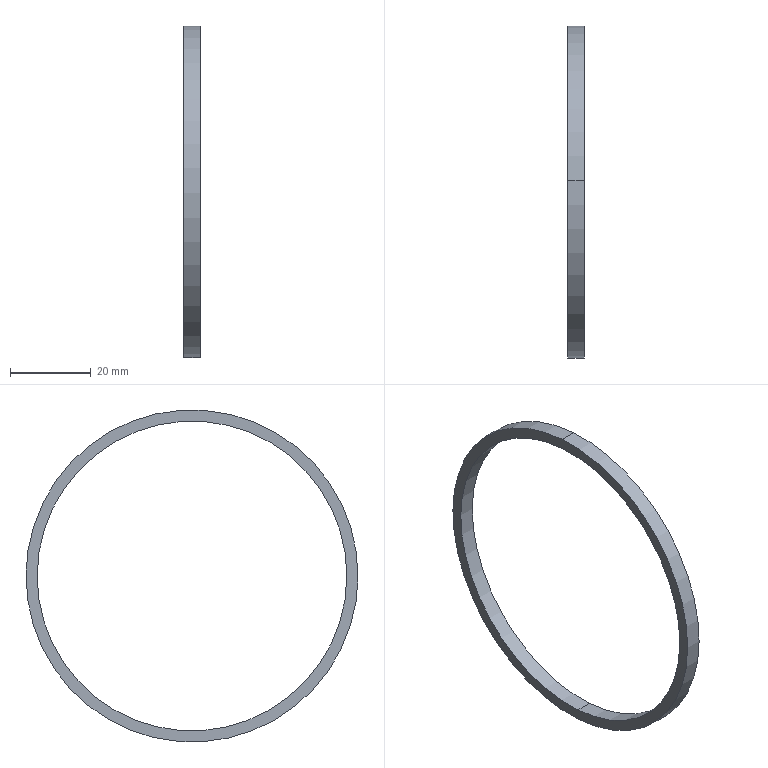Component | SolidWorks | 2018SOLIDWORKS1000000506-1 | 1 solid | 6 faces | box 4 x 82 x 82 mm | volume 2739 mm3 | cylinder 4 | plane 2 | commonest cylinder face diameters 76.5 x2 82 x2 | material 201
build123d program:
from build123d import *

# Parameters (mm, degrees)
SKETCH1_R           = 41
SKETCH1_R_2         = 38.25
BOSS_EXTRUDE1_DEPTH = 4


with BuildPart() as part:
    # Sketch1 → Boss-Extrude1 (new body)
    with BuildSketch(Plane.XY):
        Circle(SKETCH1_R)
        Circle(SKETCH1_R_2, mode=Mode.SUBTRACT)
    extrude(amount=BOSS_EXTRUDE1_DEPTH)


solid = part.part

# Placed as in the assembly
solid = solid.moved(Location((2.716, -95.825, 207.018), (0, 90, 0)))
STEP:
#1=COLOUR_RGB('',0.7922,0.8196,0.9333);
#2=FILL_AREA_STYLE_COLOUR('',#1);
#3=FILL_AREA_STYLE('',(#2));
#4=SURFACE_STYLE_FILL_AREA(#3);
#5=SURFACE_SIDE_STYLE('',(#4));
#6=SURFACE_STYLE_USAGE(.BOTH.,#5);
#7=PRESENTATION_STYLE_ASSIGNMENT((#6));
#8=CARTESIAN_POINT('',(0.2644,-3.668,9.653));
#9=VERTEX_POINT('',#8);
#10=CARTESIAN_POINT('',(0.2644,-3.878,6.648));
#11=VERTEX_POINT('',#10);
#12=CARTESIAN_POINT('',(0.2644,-3.773,8.15));
#13=DIRECTION('',(1.,0.,-0.));
#14=DIRECTION('',(-0.,-0.06975,-0.9976));
#15=AXIS2_PLACEMENT_3D('',#12,#13,#14);
#16=CIRCLE('',#15,1.506);
#17=EDGE_CURVE('',#9,#11,#16,.T.);
#18=ORIENTED_EDGE('',*,*,#17,.T.);
#19=CARTESIAN_POINT('',(0.1069,-3.878,6.648));
#20=VERTEX_POINT('',#19);
#21=CARTESIAN_POINT('',(0.2644,-3.878,6.648));
#22=DIRECTION('',(-1.,-0.,0.));
#23=VECTOR('',#22,39.37);
#24=LINE('',#21,#23);
#25=EDGE_CURVE('',#11,#20,#24,.T.);
#26=ORIENTED_EDGE('',*,*,#25,.T.);
#27=CARTESIAN_POINT('',(0.1069,-3.668,9.653));
#28=VERTEX_POINT('',#27);
#29=CARTESIAN_POINT('',(0.1069,-3.773,8.15));
#30=DIRECTION('',(1.,0.,-0.));
#31=DIRECTION('',(-0.,-0.06975,-0.9976));
#32=AXIS2_PLACEMENT_3D('',#29,#30,#31);
#33=CIRCLE('',#32,1.506);
#34=EDGE_CURVE('',#28,#20,#33,.T.);
#35=ORIENTED_EDGE('',*,*,#34,.F.);
#36=CARTESIAN_POINT('',(0.2644,-3.668,9.653));
#37=DIRECTION('',(-1.,-0.,0.));
#38=VECTOR('',#37,39.37);
#39=LINE('',#36,#38);
#40=EDGE_CURVE('',#9,#28,#39,.T.);
#41=ORIENTED_EDGE('',*,*,#40,.F.);
#42=EDGE_LOOP('',(#18,#26,#35,#41));
#43=FACE_OUTER_BOUND('',#42,.T.);
#44=CARTESIAN_POINT('',(0.2644,-3.773,8.15));
#45=DIRECTION('',(-1.,-0.,0.));
#46=DIRECTION('',(0.,0.06975,0.9976));
#47=AXIS2_PLACEMENT_3D('',#44,#45,#46);
#48=CYLINDRICAL_SURFACE('',#47,1.506);
#49=ADVANCED_FACE('',(#43),#48,.F.);
#50=CARTESIAN_POINT('',(0.2644,-3.885,6.54));
#51=VERTEX_POINT('',#50);
#52=CARTESIAN_POINT('',(0.2644,-3.66,9.761));
#53=VERTEX_POINT('',#52);
#54=CARTESIAN_POINT('',(0.2644,-3.773,8.15));
#55=DIRECTION('',(1.,0.,-0.));
#56=DIRECTION('',(-0.,-0.06975,-0.9976));
#57=AXIS2_PLACEMENT_3D('',#54,#55,#56);
#58=CIRCLE('',#57,1.614);
#59=EDGE_CURVE('',#51,#53,#58,.T.);
#60=ORIENTED_EDGE('',*,*,#59,.F.);
#61=CARTESIAN_POINT('',(0.1069,-3.885,6.54));
#62=VERTEX_POINT('',#61);
#63=CARTESIAN_POINT('',(0.2644,-3.885,6.54));
#64=DIRECTION('',(-1.,-0.,0.));
#65=VECTOR('',#64,39.37);
#66=LINE('',#63,#65);
#67=EDGE_CURVE('',#51,#62,#66,.T.);
#68=ORIENTED_EDGE('',*,*,#67,.T.);
#69=CARTESIAN_POINT('',(0.1069,-3.66,9.761));
#70=VERTEX_POINT('',#69);
#71=CARTESIAN_POINT('',(0.1069,-3.773,8.15));
#72=DIRECTION('',(1.,0.,-0.));
#73=DIRECTION('',(-0.,-0.06975,-0.9976));
#74=AXIS2_PLACEMENT_3D('',#71,#72,#73);
#75=CIRCLE('',#74,1.614);
#76=EDGE_CURVE('',#62,#70,#75,.T.);
#77=ORIENTED_EDGE('',*,*,#76,.T.);
#78=CARTESIAN_POINT('',(0.2644,-3.66,9.761));
#79=DIRECTION('',(-1.,-0.,0.));
#80=VECTOR('',#79,39.37);
#81=LINE('',#78,#80);
#82=EDGE_CURVE('',#53,#70,#81,.T.);
#83=ORIENTED_EDGE('',*,*,#82,.F.);
#84=EDGE_LOOP('',(#60,#68,#77,#83));
#85=FACE_OUTER_BOUND('',#84,.T.);
#86=CARTESIAN_POINT('',(0.2644,-3.773,8.15));
#87=DIRECTION('',(-1.,-0.,0.));
#88=DIRECTION('',(0.,0.06975,0.9976));
#89=AXIS2_PLACEMENT_3D('',#86,#87,#88);
#90=CYLINDRICAL_SURFACE('',#89,1.614);
#91=ADVANCED_FACE('',(#85),#90,.T.);
#92=CARTESIAN_POINT('',(0.2644,-3.773,8.15));
#93=DIRECTION('',(1.,0.,-0.));
#94=DIRECTION('',(-0.,-0.06975,-0.9976));
#95=AXIS2_PLACEMENT_3D('',#92,#93,#94);
#96=CIRCLE('',#95,1.614);
#97=EDGE_CURVE('',#53,#51,#96,.T.);
#98=ORIENTED_EDGE('',*,*,#97,.T.);
#99=ORIENTED_EDGE('',*,*,#59,.T.);
#100=EDGE_LOOP('',(#98,#99));
#101=FACE_OUTER_BOUND('',#100,.T.);
#102=ORIENTED_EDGE('',*,*,#17,.F.);
#103=CARTESIAN_POINT('',(0.2644,-3.773,8.15));
#104=DIRECTION('',(1.,0.,-0.));
#105=DIRECTION('',(-0.,-0.06975,-0.9976));
#106=AXIS2_PLACEMENT_3D('',#103,#104,#105);
#107=CIRCLE('',#106,1.506);
#108=EDGE_CURVE('',#11,#9,#107,.T.);
#109=ORIENTED_EDGE('',*,*,#108,.F.);
#110=EDGE_LOOP('',(#102,#109));
#111=FACE_BOUND('',#110,.T.);
#112=CARTESIAN_POINT('',(0.2644,-3.773,8.15));
#113=DIRECTION('',(1.,0.,-0.));
#114=DIRECTION('',(-0.,-0.06975,-0.9976));
#115=AXIS2_PLACEMENT_3D('',#112,#113,#114);
#116=PLANE('',#115);
#117=ADVANCED_FACE('',(#101,#111),#116,.T.);
#118=CARTESIAN_POINT('',(0.1069,-3.773,8.15));
#119=DIRECTION('',(1.,0.,-0.));
#120=DIRECTION('',(-0.,-0.06975,-0.9976));
#121=AXIS2_PLACEMENT_3D('',#118,#119,#120);
#122=CIRCLE('',#121,1.614);
#123=EDGE_CURVE('',#70,#62,#122,.T.);
#124=ORIENTED_EDGE('',*,*,#123,.F.);
#125=ORIENTED_EDGE('',*,*,#76,.F.);
#126=EDGE_LOOP('',(#124,#125));
#127=FACE_OUTER_BOUND('',#126,.T.);
#128=ORIENTED_EDGE('',*,*,#34,.T.);
#129=CARTESIAN_POINT('',(0.1069,-3.773,8.15));
#130=DIRECTION('',(1.,0.,-0.));
#131=DIRECTION('',(-0.,-0.06975,-0.9976));
#132=AXIS2_PLACEMENT_3D('',#129,#130,#131);
#133=CIRCLE('',#132,1.506);
#134=EDGE_CURVE('',#20,#28,#133,.T.);
#135=ORIENTED_EDGE('',*,*,#134,.T.);
#136=EDGE_LOOP('',(#128,#135));
#137=FACE_BOUND('',#136,.T.);
#138=CARTESIAN_POINT('',(0.1069,-3.773,8.15));
#139=DIRECTION('',(1.,0.,-0.));
#140=DIRECTION('',(-0.,-0.06975,-0.9976));
#141=AXIS2_PLACEMENT_3D('',#138,#139,#140);
#142=PLANE('',#141);
#143=ADVANCED_FACE('',(#127,#137),#142,.F.);
#144=ORIENTED_EDGE('',*,*,#67,.F.);
#145=ORIENTED_EDGE('',*,*,#97,.F.);
#146=ORIENTED_EDGE('',*,*,#82,.T.);
#147=ORIENTED_EDGE('',*,*,#123,.T.);
#148=EDGE_LOOP('',(#144,#145,#146,#147));
#149=FACE_OUTER_BOUND('',#148,.T.);
#150=CARTESIAN_POINT('',(0.2644,-3.773,8.15));
#151=DIRECTION('',(-1.,-0.,0.));
#152=DIRECTION('',(0.,0.06975,0.9976));
#153=AXIS2_PLACEMENT_3D('',#150,#151,#152);
#154=CYLINDRICAL_SURFACE('',#153,1.614);
#155=ADVANCED_FACE('',(#149),#154,.T.);
#156=ORIENTED_EDGE('',*,*,#25,.F.);
#157=ORIENTED_EDGE('',*,*,#108,.T.);
#158=ORIENTED_EDGE('',*,*,#40,.T.);
#159=ORIENTED_EDGE('',*,*,#134,.F.);
#160=EDGE_LOOP('',(#156,#157,#158,#159));
#161=FACE_OUTER_BOUND('',#160,.T.);
#162=CARTESIAN_POINT('',(0.2644,-3.773,8.15));
#163=DIRECTION('',(-1.,-0.,0.));
#164=DIRECTION('',(0.,0.06975,0.9976));
#165=AXIS2_PLACEMENT_3D('',#162,#163,#164);
#166=CYLINDRICAL_SURFACE('',#165,1.506);
#167=ADVANCED_FACE('',(#161),#166,.F.);
#168=CLOSED_SHELL('',(#49,#91,#117,#143,#155,#167));
#169=MANIFOLD_SOLID_BREP('',#168);
#170=STYLED_ITEM('',(#7),#169);
#171=(LENGTH_UNIT()NAMED_UNIT(*)SI_UNIT($,.METRE.));
#172=LENGTH_MEASURE_WITH_UNIT(LENGTH_MEASURE(0.0254),#171);
#173=DIMENSIONAL_EXPONENTS(1.,0.,0.,0.,0.,0.,0.);
#174=(CONVERSION_BASED_UNIT('',#172)LENGTH_UNIT()NAMED_UNIT(#173));
#175=UNCERTAINTY_MEASURE_WITH_UNIT(LENGTH_MEASURE(0.00001),#174,'','');
#176=(NAMED_UNIT(*)PLANE_ANGLE_UNIT()SI_UNIT($,.RADIAN.));
#177=(NAMED_UNIT(*)SI_UNIT($,.STERADIAN.)SOLID_ANGLE_UNIT());
#178=(GEOMETRIC_REPRESENTATION_CONTEXT(3)GLOBAL_UNCERTAINTY_ASSIGNED_CONTEXT((#175))GLOBAL_UNIT_ASSIGNED_CONTEXT((#174,#176,#177))REPRESENTATION_CONTEXT('',''));
#179=MECHANICAL_DESIGN_GEOMETRIC_PRESENTATION_REPRESENTATION('',(#170),#178);
#180=PRESENTATION_LAYER_ASSIGNMENT('','',(#170));
#181=CARTESIAN_POINT('',(0.,0.,0.));
#182=DIRECTION('',(0.,0.,1.));
#183=DIRECTION('',(1.,0.,0.));
#184=AXIS2_PLACEMENT_3D('',#181,#182,#183);
#185=(LENGTH_UNIT()NAMED_UNIT(*)SI_UNIT($,.METRE.));
#186=LENGTH_MEASURE_WITH_UNIT(LENGTH_MEASURE(0.0254),#185);
#187=DIMENSIONAL_EXPONENTS(1.,0.,0.,0.,0.,0.,0.);
#188=(CONVERSION_BASED_UNIT('',#186)LENGTH_UNIT()NAMED_UNIT(#187));
#189=UNCERTAINTY_MEASURE_WITH_UNIT(LENGTH_MEASURE(0.00001),#188,'','');
#190=(NAMED_UNIT(*)PLANE_ANGLE_UNIT()SI_UNIT($,.RADIAN.));
#191=(NAMED_UNIT(*)SI_UNIT($,.STERADIAN.)SOLID_ANGLE_UNIT());
#192=(GEOMETRIC_REPRESENTATION_CONTEXT(3)GLOBAL_UNCERTAINTY_ASSIGNED_CONTEXT((#189))GLOBAL_UNIT_ASSIGNED_CONTEXT((#188,#190,#191))REPRESENTATION_CONTEXT('',''));
#193=ADVANCED_BREP_SHAPE_REPRESENTATION('',(#169,#184),#192);